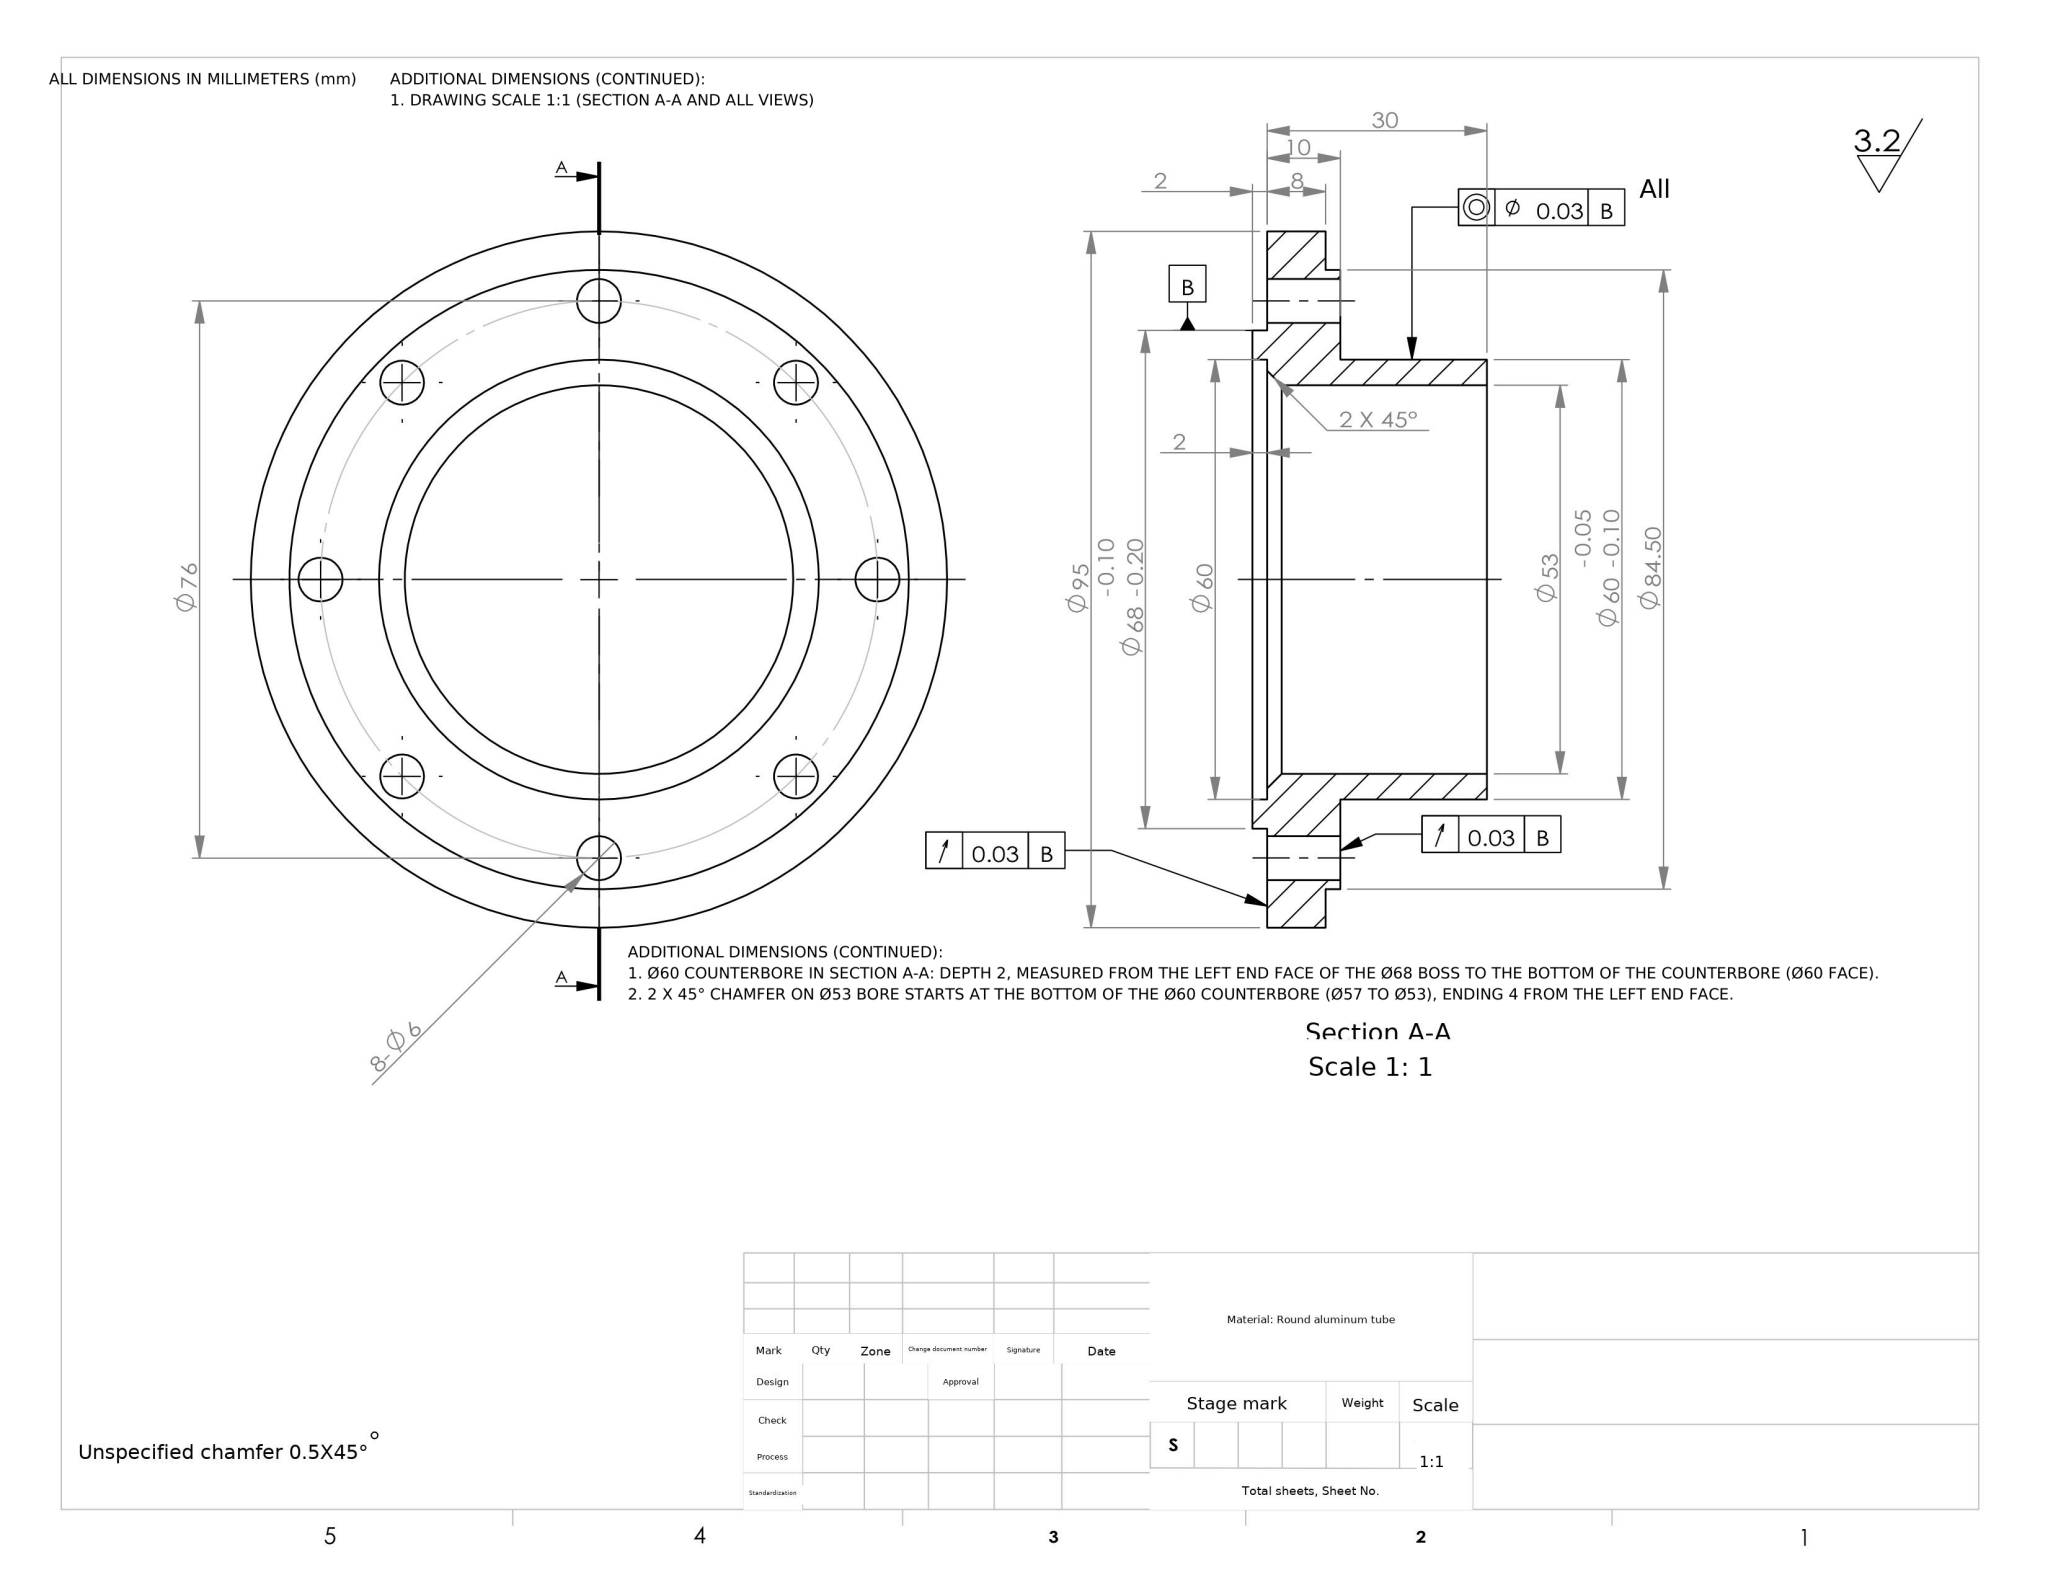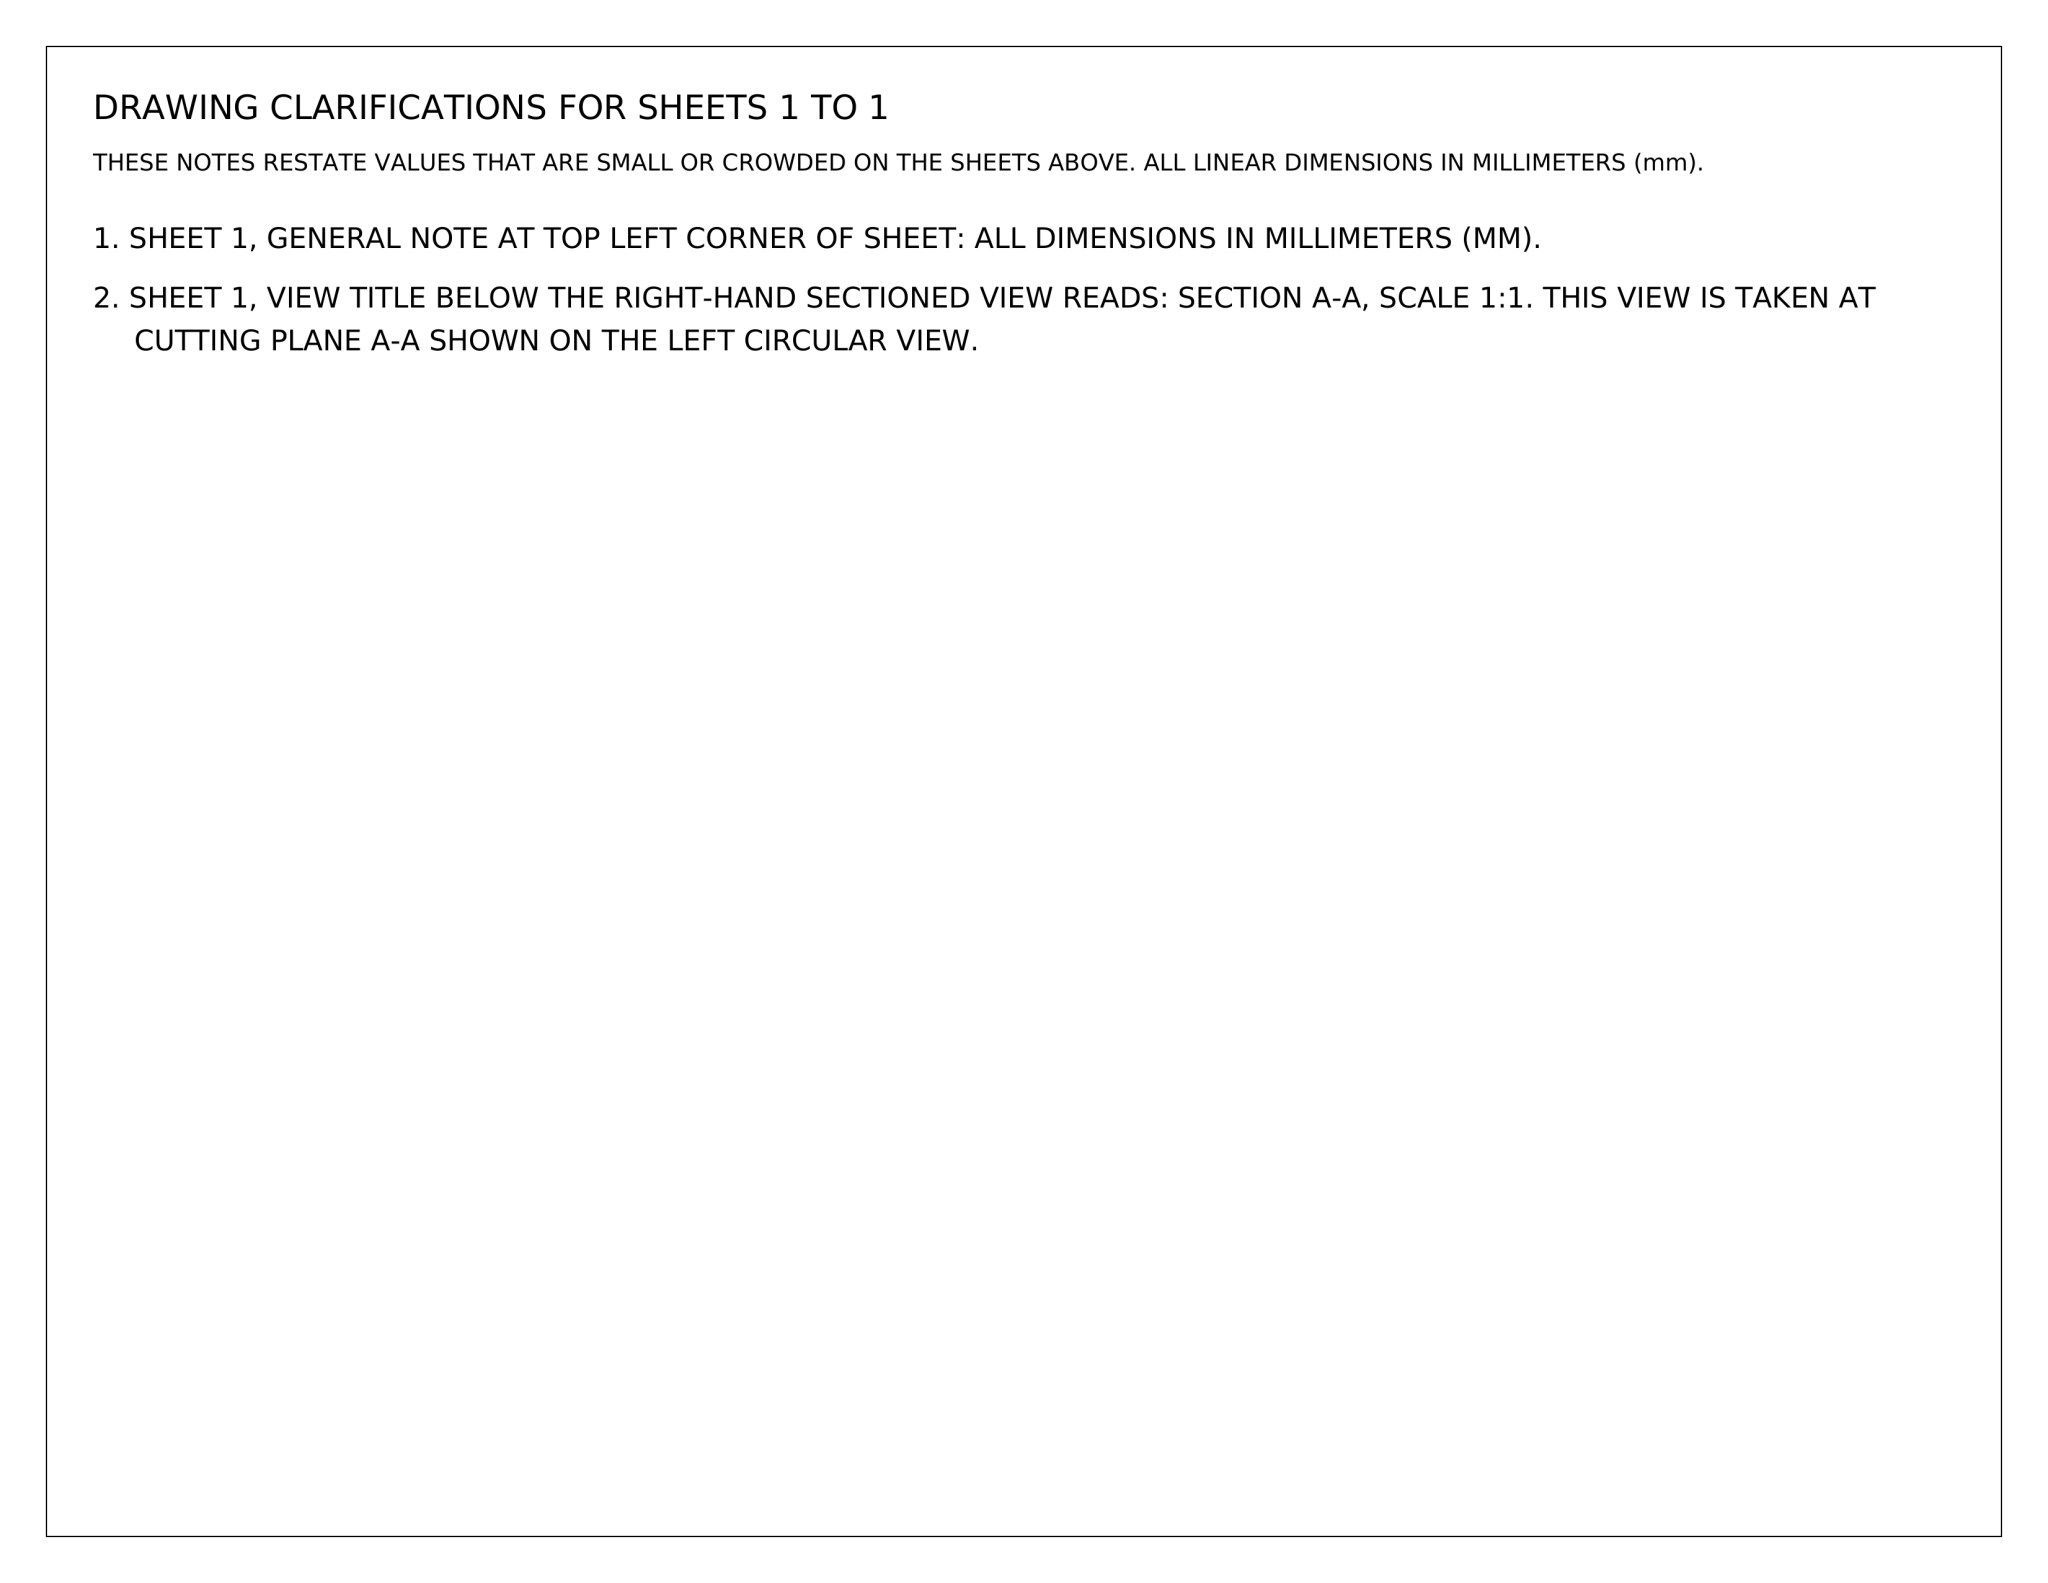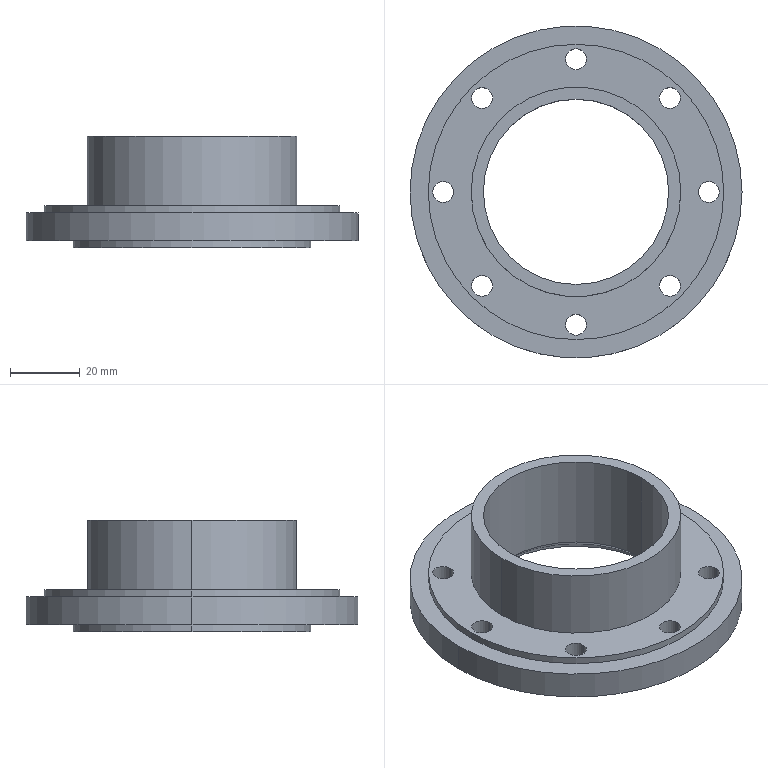Part | NX | mm | 1 solid | 36 faces | box 95 x 95 x 32 mm | volume 57290 mm3 | cylinder 28 | plane 6 | cone 2 | commonest cylinder face diameters 6 x16 60 x4 84.5 x2 68 x2 53 x2 95 x2